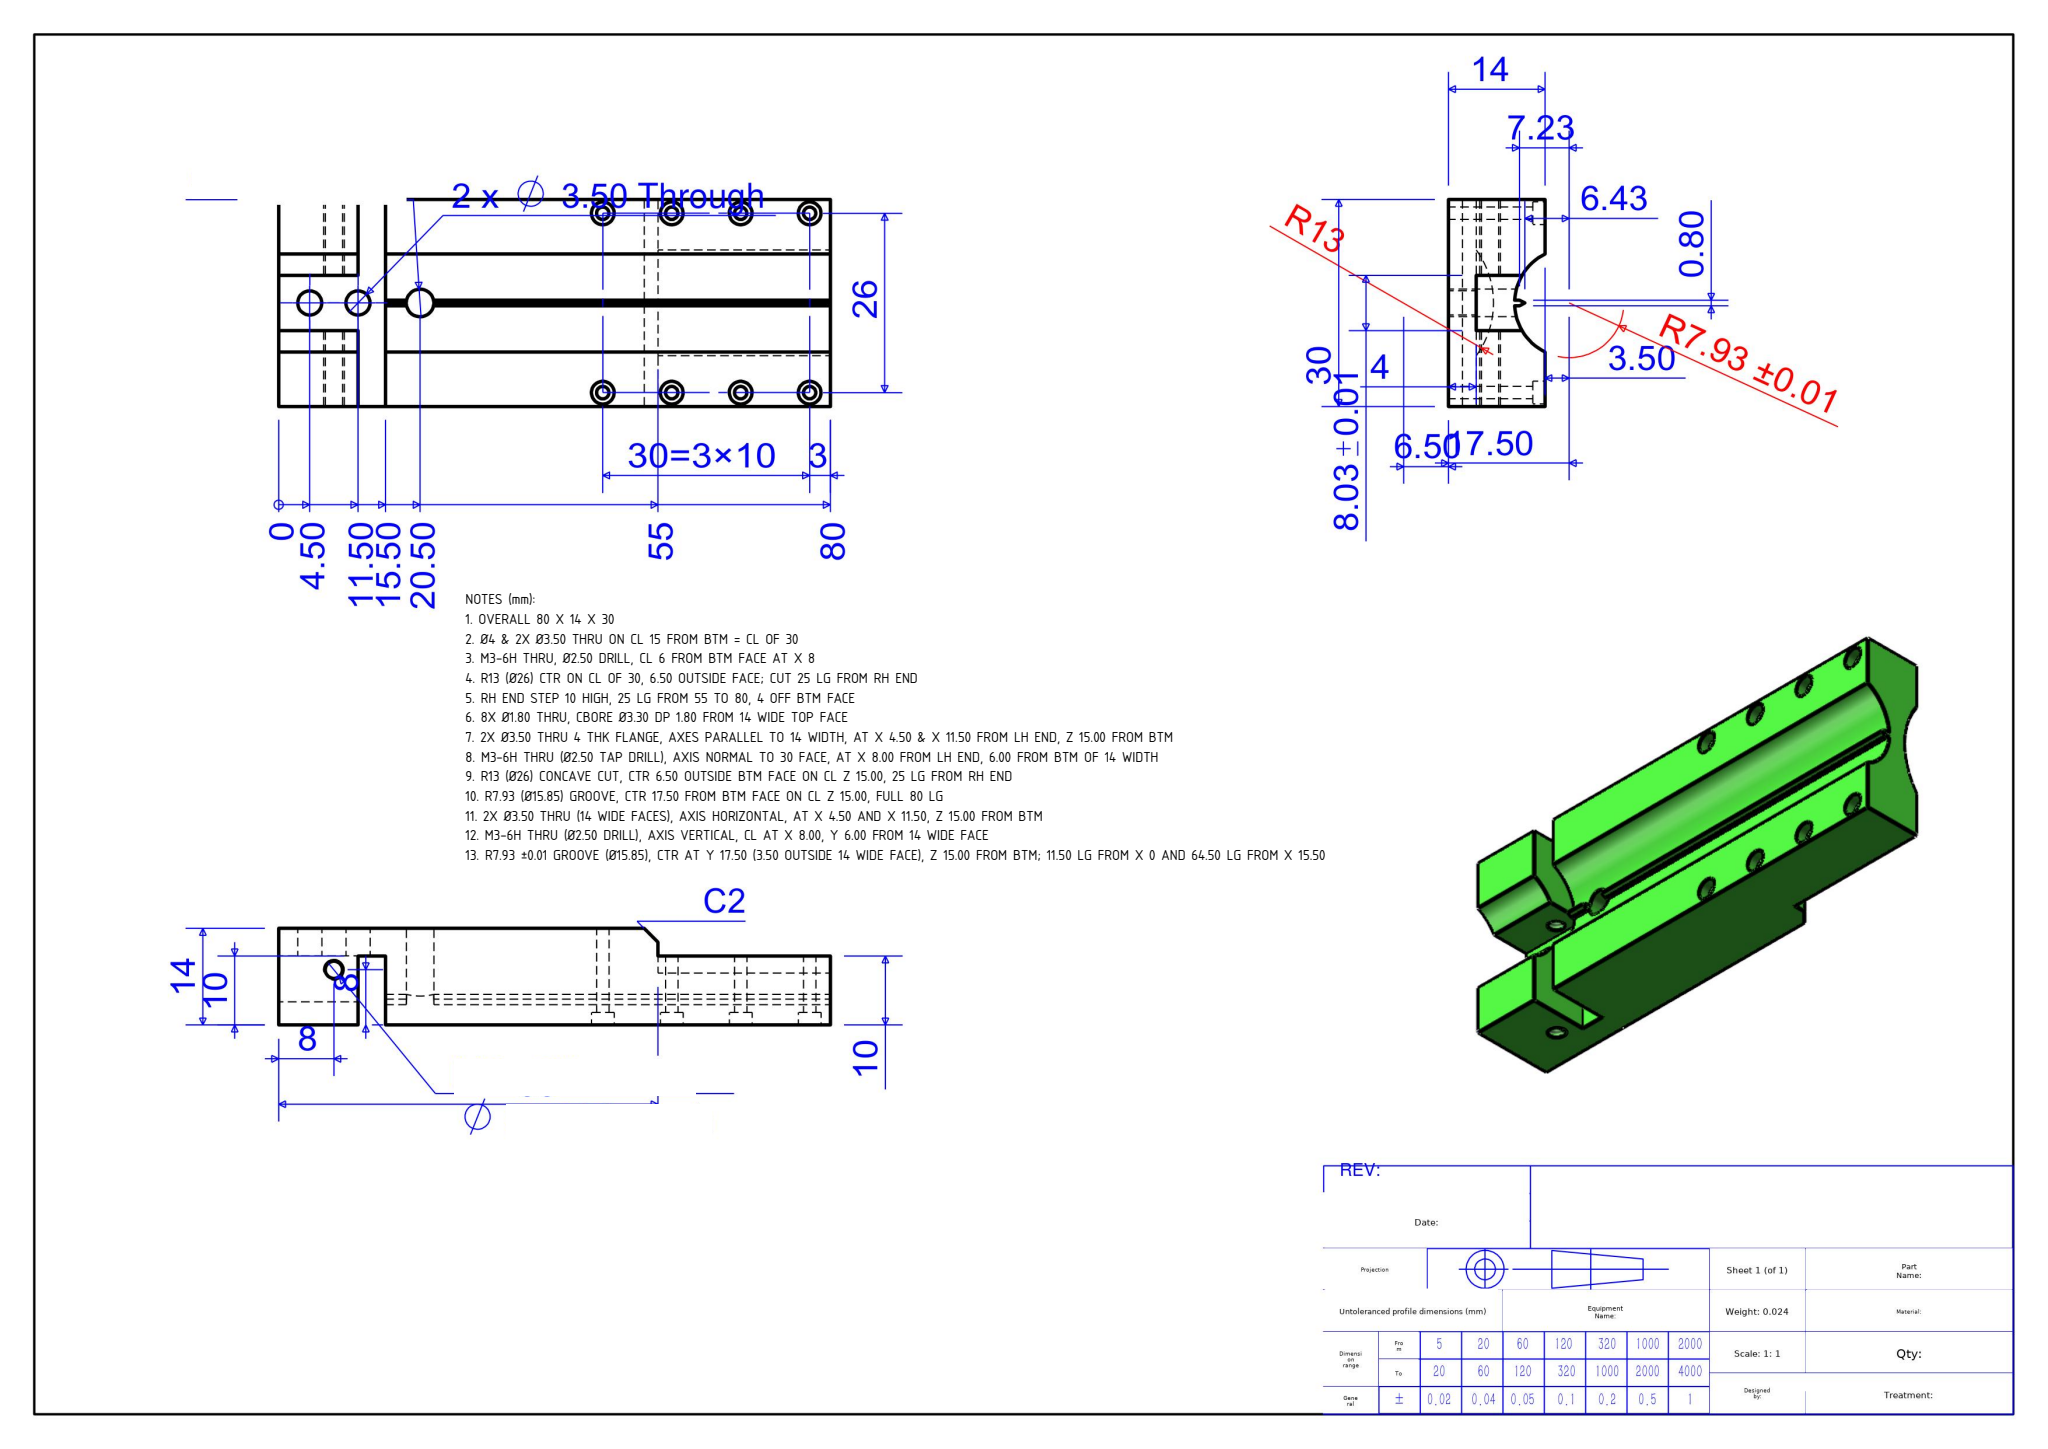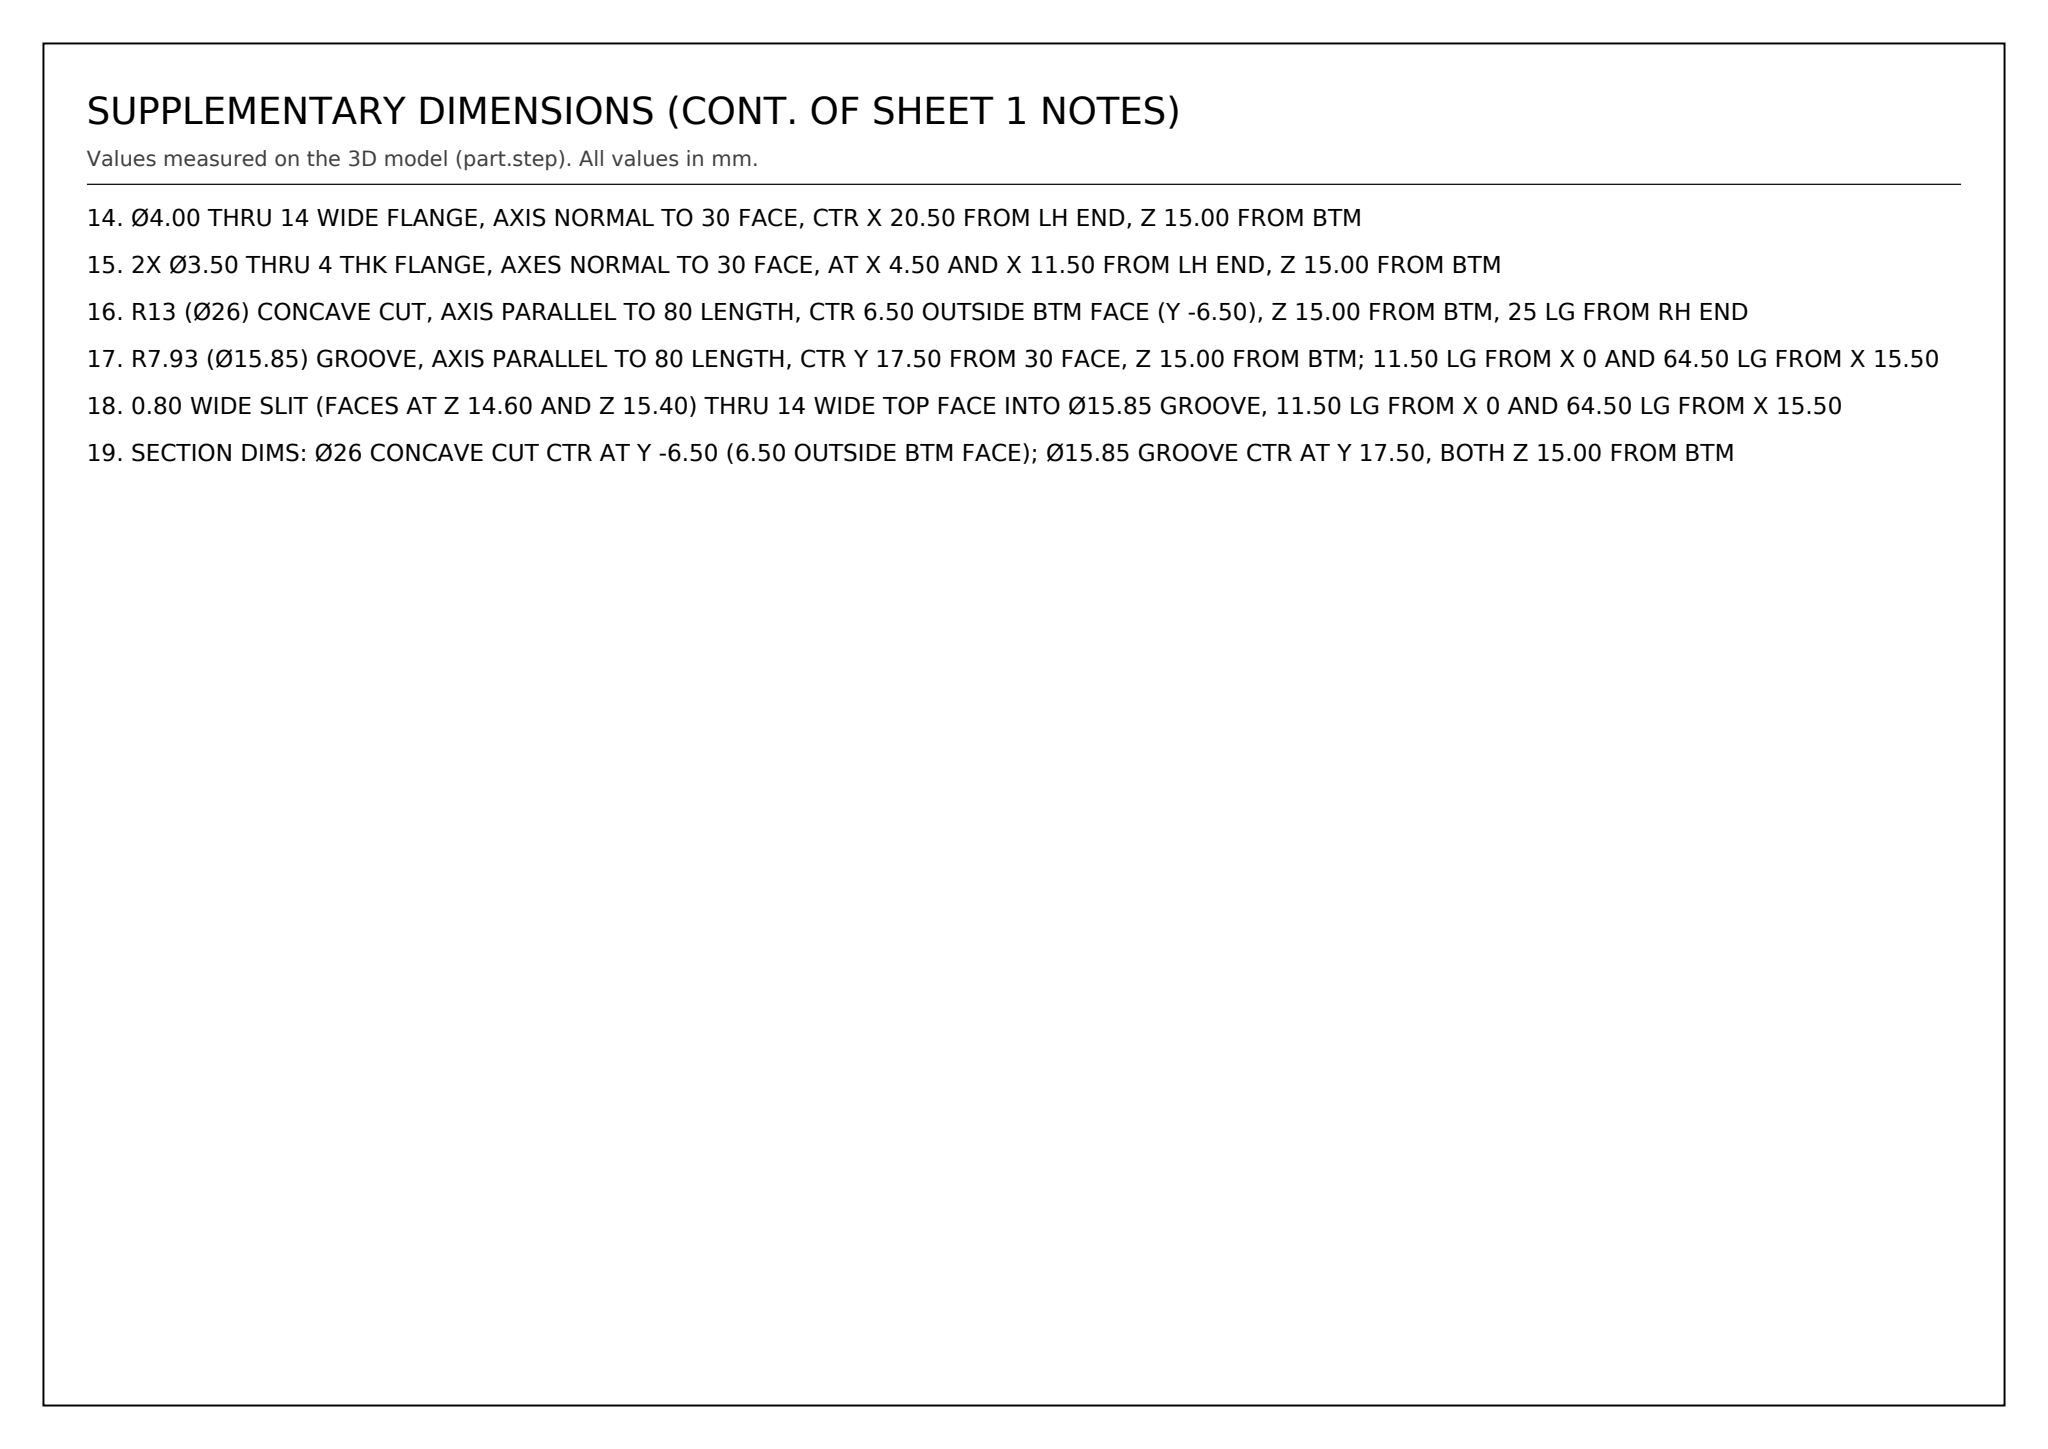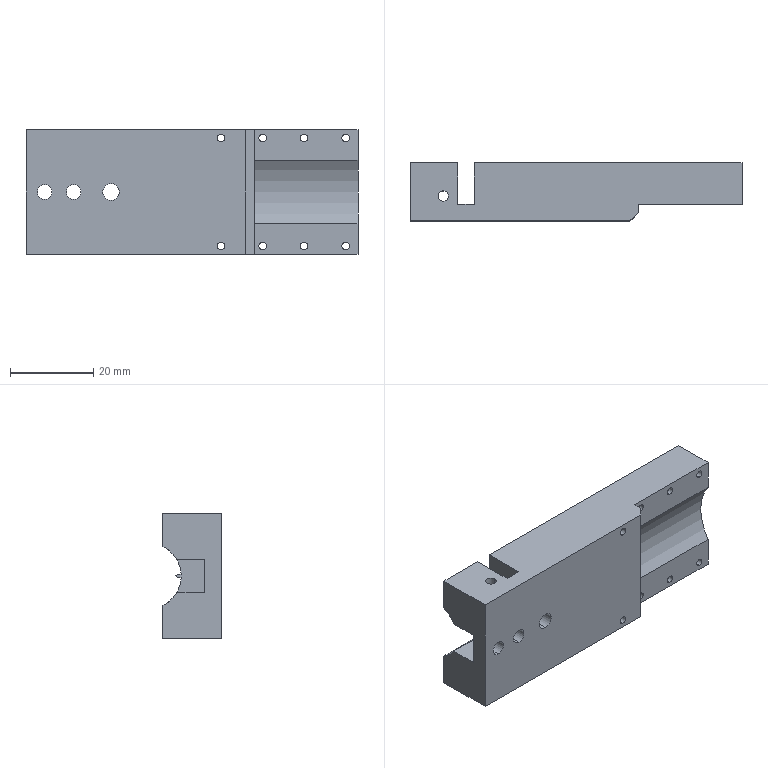Part | SolidWorks | mm | 1 solid | 82 faces | box 80 x 14 x 30 mm | volume 24154 mm3 | cylinder 47 | plane 35 | commonest cylinder face diameters 3.3 x16 1.8 x16 2.5 x4 3.5 x4 15.85 x4 4 x2 26 x1
Drawing notes:
OVERALL 80 X 14 X 30 | from the solid: bbox_xyz 80.0 x 14.0 x 30.0
Ø4 & 2X Ø3.50 THRU ON CL 15 FROM BTM = CL OF 30 | from the solid: Ø4 cyl axis y at (x=20.5, z=15.0); Ø3.5 cyls axis y at (x=4.5 & 11.5, z=15.0); bbox z=30
M3-6H THRU, Ø2.50 DRILL, CL 6 FROM BTM FACE AT X 8 | from the solid: Ø2.5 cyl axis z at (x=8.0, y=6.0), length 10.99
R13 (Ø26) CTR ON CL OF 30, 6.50 OUTSIDE FACE; CUT 25 LG FROM RH END | from the solid: Ø26 cyl axis x at (y=-6.5, z=15.0), length 25 -> x=55 to 80
RH END STEP 10 HIGH, 25 LG FROM 55 TO 80, 4 OFF BTM FACE | from the solid: planes x=55 and x=80 (25 lg); plane y=4.0 with bbox y=14 -> 10 remaining
8X Ø1.80 THRU, CBORE Ø3.30 DP 1.80 FROM 14 WIDE TOP FACE | from the solid: Ø1.8 y-axis holes at x=47,57,67,77 / z=2,28 (len 12.2 & 8.2) each with Ø3.3 c'bore len 1.8 starting at y=14 face (c'bore floor plane y=12.2)
2X Ø3.50 THRU 4 THK FLANGE, AXES PARALLEL TO 14 WIDTH, AT X 4.50 & X 11.50 FROM LH END, Z 15.00 FROM BTM | from the solid: cylinders [3.5,"y",[4.5,null,15.0],4.0] and [3.5,"y",[11.5,null,15.0],4.0]
M3-6H THRU (Ø2.50 TAP DRILL), AXIS NORMAL TO 30 FACE, AT X 8.00 FROM LH END, 6.00 FROM BTM OF 14 WIDTH | from the solid: cylinder [2.5,"z",[8.0,6.0,null],10.99]
R13 (Ø26) CONCAVE CUT, CTR 6.50 OUTSIDE BTM FACE ON CL Z 15.00, 25 LG FROM RH END | from the solid: cylinder [26.0,"x",[null,-6.5,15.0],25.0]
R7.93 (Ø15.85) GROOVE, CTR 17.50 FROM BTM FACE ON CL Z 15.00, FULL 80 LG | from the solid: cylinders [15.85,"x",[null,17.5,15.0],11.5] and [15.85,"x",[null,17.5,15.0],64.5]
2X Ø3.50 THRU (14 WIDE FACES), AXIS HORIZONTAL, AT X 4.50 AND X 11.50, Z 15.00 FROM BTM | from the solid: cylinders [3.5,"y",[4.5,null,15.0],4.0] and [3.5,"y",[11.5,null,15.0],4.0]
M3-6H THRU (Ø2.50 DRILL), AXIS VERTICAL, CL AT X 8.00, Y 6.00 FROM 14 WIDE FACE | from the solid: cylinders [2.5,"z",[8.0,6.0,null],10.99]
R7.93 ±0.01 GROOVE (Ø15.85), CTR AT Y 17.50 (3.50 OUTSIDE 14 WIDE FACE), Z 15.00 FROM BTM; 11.50 LG FROM X 0 AND 64.50 LG FROM X 15.50 | from the solid: cylinders [15.85,"x",[null,17.5,15.0],11.5] and [15.85,"x",[null,17.5,15.0],64.5]
Ø4.00 THRU 14 WIDE FLANGE, AXIS NORMAL TO 30 FACE, CTR X 20.50 FROM LH END, Z 15.00 FROM BTM | from the solid: cylinders: [4.0,'y',[20.5,null,15.0],11.08]
2X Ø3.50 THRU 4 THK FLANGE, AXES NORMAL TO 30 FACE, AT X 4.50 AND X 11.50 FROM LH END, Z 15.00 FROM BTM | from the solid: cylinders: [3.5,'y',[4.5,null,15.0],4.0] and [3.5,'y',[11.5,null,15.0],4.0]
R13 (Ø26) CONCAVE CUT, AXIS PARALLEL TO 80 LENGTH, CTR 6.50 OUTSIDE BTM FACE (Y -6.50), Z 15.00 FROM BTM, 25 LG FROM RH END | from the solid: cylinders: [26.0,'x',[null,-6.5,15.0],25.0]
R7.93 (Ø15.85) GROOVE, AXIS PARALLEL TO 80 LENGTH, CTR Y 17.50 FROM 30 FACE, Z 15.00 FROM BTM; 11.50 LG FROM X 0 AND 64.50 LG FROM X 15.50 | from the solid: cylinders: [15.85,'x',[null,17.5,15.0],11.5] and [15.85,'x',[null,17.5,15.0],64.5]
0.80 WIDE SLIT (FACES AT Z 14.60 AND Z 15.40) THRU 14 WIDE TOP FACE INTO Ø15.85 GROOVE, 11.50 LG FROM X 0 AND 64.50 LG FROM X 15.50 | from the solid: axis_planes z=14.6 (2) and z=15.4 (2), matching the two Ø15.85 x-axis groove segments of length 11.50 (from x 0) and 64.50 (from x 15.50)
SECTION DIMS: Ø26 CONCAVE CUT CTR AT Y -6.50 (6.50 OUTSIDE BTM FACE); Ø15.85 GROOVE CTR AT Y 17.50, BOTH Z 15.00 FROM BTM | from the solid: cylinders [26.0,'x',[null,-6.5,15.0],25.0] and [15.85,'x',[null,17.5,15.0],...]
build123d program:
from build123d import *

# Parameters (mm, degrees)
SKETCH1_W                                         = 80
SKETCH1_H                                         = 30
BOSS_EXTRUDE1_DEPTH                               = 14
SKETCH8_W                                         = 23
SKETCH8_H                                         = 8.03
SKETCH8_W_2                                       = 4
SKETCH8_H_2                                       = 30
CUT_EXTRUDE3_DEPTH                                = 10
SKETCH9_R                                         = 7.925
CUT_EXTRUDE4_DEPTH                                = 83.589
F_3_5_3_5_DIAMETER_HOLE1_D                        = 3.5
SKETCH12_R                                        = 13
CUT_EXTRUDE5_DEPTH                                = 25
SKETCH13_W                                        = 30
SKETCH13_H                                        = 6.546
CUT_EXTRUDE6_DEPTH                                = 25
CHAMFER1_SIZE                                     = 2
BOSS_EXTRUDE2_START                               = -64.5
BOSS_EXTRUDE2_DEPTH                               = 64.5
F_1_0_1_DIAMETER_HOLE1_D                          = 4
M3_TAPPED_HOLE1_D                                 = 2.5
M1_6_HEX_SOCKET_HEAD_CAP_SCREW_CBORE1_D           = 1.8
M1_6_HEX_SOCKET_HEAD_CAP_SCREW_CBORE1_DEPTH       = 20
M1_6_HEX_SOCKET_HEAD_CAP_SCREW_CBORE1_CBORE_D     = 3.3
M1_6_HEX_SOCKET_HEAD_CAP_SCREW_CBORE1_CBORE_DEPTH = 1.8
M1_6_HEX_SOCKET_HEAD_CAP_SCREW_CBORE1_TIP         = 0.5408


with BuildPart() as part:
    # Sketch1 → Boss-Extrude1 (new body)
    with BuildSketch(Plane(origin=(0, 0, 0), x_dir=(1, 0, 0), z_dir=(0, 1, 0))):
        Rectangle(SKETCH1_W, SKETCH1_H)
    extrude(amount=BOSS_EXTRUDE1_DEPTH)

    # Sketch8 → Cut-Extrude3 (cut)
    with BuildSketch(Plane(origin=(0, 14, 0), x_dir=(1, 0, 0), z_dir=(0, 1, 0))):
        with Locations((-40, 0)):
            Rectangle(SKETCH8_W, SKETCH8_H)
        with Locations((-26.5, 0)):
            Rectangle(SKETCH8_W_2, SKETCH8_H_2)
    extrude(amount=-CUT_EXTRUDE3_DEPTH, mode=Mode.SUBTRACT)

    # Sketch9 → Cut-Extrude4 (cut, through all)
    with BuildSketch(Plane(origin=(40, 0, 0), x_dir=(0, 0, -1), z_dir=(1, 0, 0))):
        with Locations((0, 17.5)):
            Circle(SKETCH9_R)
    extrude(amount=-CUT_EXTRUDE4_DEPTH, mode=Mode.SUBTRACT)

    # 3.5 _3.5_ Diameter Hole1 (through all)
    with Locations(Plane(origin=(0, 0, 0), x_dir=(-1, 0, 0), z_dir=(0, -1, 0))):
        with Locations((35.5, 0), (28.5, 0)):
            Hole(F_3_5_3_5_DIAMETER_HOLE1_D / 2)

    # Sketch12 → Cut-Extrude5 (cut)
    with BuildSketch(Plane(origin=(40, 0, 0), x_dir=(0, 0, -1), z_dir=(1, 0, 0))):
        with Locations((0, -6.5)):
            Circle(SKETCH12_R)
    extrude(amount=-CUT_EXTRUDE5_DEPTH, mode=Mode.SUBTRACT)

    # Sketch13 → Cut-Extrude6 (cut)
    with BuildSketch(Plane(origin=(40, 0, 0), x_dir=(0, 0, -1), z_dir=(1, 0, 0))):
        with Locations((0, 0.727)):
            Rectangle(SKETCH13_W, SKETCH13_H)
    extrude(amount=-CUT_EXTRUDE6_DEPTH, mode=Mode.SUBTRACT)

    # Chamfer1
    chamfer1_edges = [part.edges().sort_by_distance(p)[0] for p in [
        (15, 0, 0),
    ]]
    chamfer(chamfer1_edges, length=CHAMFER1_SIZE)

    # Sketch14 → Boss-Extrude2 (add)
    with BuildSketch(Plane(origin=(40, 0, 0), x_dir=(0, 0, -1), z_dir=(1, 0, 0)).offset(BOSS_EXTRUDE2_START)):
        Polygon((-0.4, 9.575), (0.4, 9.575), (0.4, 10.275), (0, 11.075), (-0.4, 10.275), align=None)
    extrude(amount=BOSS_EXTRUDE2_DEPTH)

    # 1.0 _1_ Diameter Hole1 (through all)
    with Locations(Plane(origin=(0, 0, 0), x_dir=(-1, 0, 0), z_dir=(0, -1, 0))):
        with Locations((19.5, 0)):
            Hole(F_1_0_1_DIAMETER_HOLE1_D / 2)

    # M3 Tapped Hole1 (through all)
    with Locations(Plane.XY.offset(15)):
        with Locations((-32, 6)):
            Hole(M3_TAPPED_HOLE1_D / 2)

    # M1.6 Hex Socket Head Cap Screw CBORE1
    with Locations(Plane(origin=(0, 14, 0), x_dir=(1, 0, 0), z_dir=(0, 1, 0))):
        with Locations((37, -13), (27, -13), (27, 13), (37, 13), (17, -13), (7, -13), (7, 13), (17, 13)):
            CounterBoreHole(M1_6_HEX_SOCKET_HEAD_CAP_SCREW_CBORE1_D / 2, M1_6_HEX_SOCKET_HEAD_CAP_SCREW_CBORE1_CBORE_D / 2, M1_6_HEX_SOCKET_HEAD_CAP_SCREW_CBORE1_CBORE_DEPTH, depth=M1_6_HEX_SOCKET_HEAD_CAP_SCREW_CBORE1_DEPTH)
            with Locations((0, 0, -(M1_6_HEX_SOCKET_HEAD_CAP_SCREW_CBORE1_DEPTH + M1_6_HEX_SOCKET_HEAD_CAP_SCREW_CBORE1_TIP / 2))):  # 118° drill point
                Cone(0, M1_6_HEX_SOCKET_HEAD_CAP_SCREW_CBORE1_D / 2, M1_6_HEX_SOCKET_HEAD_CAP_SCREW_CBORE1_TIP, mode=Mode.SUBTRACT)


solid = part.part